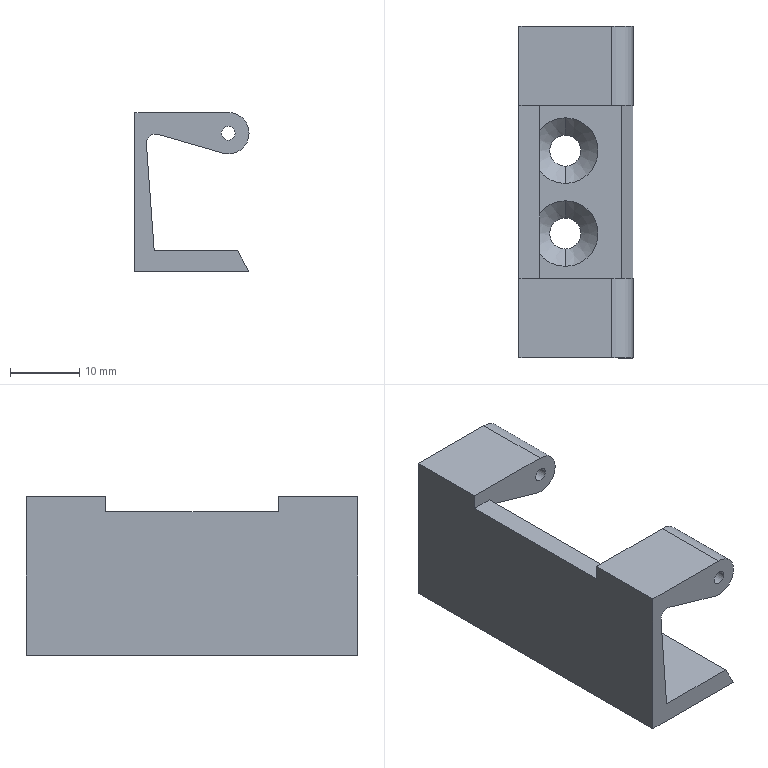Component | SolidWorks | CL201-M6-1-4 | 1 solid | 32 faces | box 16.5 x 48 x 23 mm | volume 5458 mm3 | plane 15 | cylinder 13 | cone 4 | commonest cylinder face diameters 4.5 x4 2 x4 6 x4 2.707 x1
STEP:
#1=COLOUR_RGB('',0.7922,0.8196,0.9333);
#2=FILL_AREA_STYLE_COLOUR('',#1);
#3=FILL_AREA_STYLE('',(#2));
#4=SURFACE_STYLE_FILL_AREA(#3);
#5=SURFACE_SIDE_STYLE('',(#4));
#6=SURFACE_STYLE_USAGE(.BOTH.,#5);
#7=PRESENTATION_STYLE_ASSIGNMENT((#6));
#8=CARTESIAN_POINT('',(12.006,-1.803,15.275));
#9=VERTEX_POINT('',#8);
#10=CARTESIAN_POINT('',(12.006,-1.626,15.275));
#11=VERTEX_POINT('',#10);
#12=CARTESIAN_POINT('',(12.006,-1.714,15.275));
#13=DIRECTION('',(-0.,-0.,1.));
#14=DIRECTION('',(0.,-1.,0.));
#15=AXIS2_PLACEMENT_3D('',#12,#13,#14);
#16=CIRCLE('',#15,0.08858);
#17=EDGE_CURVE('',#9,#11,#16,.T.);
#18=ORIENTED_EDGE('',*,*,#17,.F.);
#19=CARTESIAN_POINT('',(12.006,-1.901,15.373));
#20=VERTEX_POINT('',#19);
#21=CARTESIAN_POINT('',(12.006,-1.803,15.275));
#22=DIRECTION('',(-0.,-0.7071,0.7071));
#23=VECTOR('',#22,39.37);
#24=LINE('',#21,#23);
#25=EDGE_CURVE('',#9,#20,#24,.T.);
#26=ORIENTED_EDGE('',*,*,#25,.T.);
#27=CARTESIAN_POINT('',(12.006,-1.527,15.373));
#28=VERTEX_POINT('',#27);
#29=CARTESIAN_POINT('',(12.006,-1.714,15.373));
#30=DIRECTION('',(0.,0.,-1.));
#31=DIRECTION('',(0.,-1.,0.));
#32=AXIS2_PLACEMENT_3D('',#29,#30,#31);
#33=CIRCLE('',#32,0.187);
#34=EDGE_CURVE('',#28,#20,#33,.T.);
#35=ORIENTED_EDGE('',*,*,#34,.F.);
#36=CARTESIAN_POINT('',(12.006,-1.626,15.275));
#37=DIRECTION('',(-0.,0.7071,0.7071));
#38=VECTOR('',#37,39.37);
#39=LINE('',#36,#38);
#40=EDGE_CURVE('',#11,#28,#39,.T.);
#41=ORIENTED_EDGE('',*,*,#40,.F.);
#42=EDGE_LOOP('',(#18,#26,#35,#41));
#43=FACE_OUTER_BOUND('',#42,.T.);
#44=CARTESIAN_POINT('',(12.006,-1.714,15.275));
#45=DIRECTION('',(-0.,-0.,1.));
#46=DIRECTION('',(0.,1.,0.));
#47=AXIS2_PLACEMENT_3D('',#44,#45,#46);
#48=CONICAL_SURFACE('',#47,0.08858,0.7854);
#49=ADVANCED_FACE('',(#43),#48,.F.);
#50=CARTESIAN_POINT('',(12.006,-1.33,15.275));
#51=VERTEX_POINT('',#50);
#52=CARTESIAN_POINT('',(12.006,-1.153,15.275));
#53=VERTEX_POINT('',#52);
#54=CARTESIAN_POINT('',(12.006,-1.242,15.275));
#55=DIRECTION('',(-0.,-0.,1.));
#56=DIRECTION('',(0.,-1.,0.));
#57=AXIS2_PLACEMENT_3D('',#54,#55,#56);
#58=CIRCLE('',#57,0.08858);
#59=EDGE_CURVE('',#51,#53,#58,.T.);
#60=ORIENTED_EDGE('',*,*,#59,.F.);
#61=CARTESIAN_POINT('',(12.006,-1.429,15.373));
#62=VERTEX_POINT('',#61);
#63=CARTESIAN_POINT('',(12.006,-1.33,15.275));
#64=DIRECTION('',(-0.,-0.7071,0.7071));
#65=VECTOR('',#64,39.37);
#66=LINE('',#63,#65);
#67=EDGE_CURVE('',#51,#62,#66,.T.);
#68=ORIENTED_EDGE('',*,*,#67,.T.);
#69=CARTESIAN_POINT('',(12.006,-1.055,15.373));
#70=VERTEX_POINT('',#69);
#71=CARTESIAN_POINT('',(12.006,-1.242,15.373));
#72=DIRECTION('',(0.,0.,-1.));
#73=DIRECTION('',(0.,-1.,0.));
#74=AXIS2_PLACEMENT_3D('',#71,#72,#73);
#75=CIRCLE('',#74,0.187);
#76=EDGE_CURVE('',#70,#62,#75,.T.);
#77=ORIENTED_EDGE('',*,*,#76,.F.);
#78=CARTESIAN_POINT('',(12.006,-1.153,15.275));
#79=DIRECTION('',(-0.,0.7071,0.7071));
#80=VECTOR('',#79,39.37);
#81=LINE('',#78,#80);
#82=EDGE_CURVE('',#53,#70,#81,.T.);
#83=ORIENTED_EDGE('',*,*,#82,.F.);
#84=EDGE_LOOP('',(#60,#68,#77,#83));
#85=FACE_OUTER_BOUND('',#84,.T.);
#86=CARTESIAN_POINT('',(12.006,-1.242,15.275));
#87=DIRECTION('',(-0.,-0.,1.));
#88=DIRECTION('',(0.,1.,0.));
#89=AXIS2_PLACEMENT_3D('',#86,#87,#88);
#90=CONICAL_SURFACE('',#89,0.08858,0.7854);
#91=ADVANCED_FACE('',(#85),#90,.F.);
#92=CARTESIAN_POINT('',(12.006,-1.153,15.255));
#93=VERTEX_POINT('',#92);
#94=CARTESIAN_POINT('',(12.006,-1.33,15.255));
#95=VERTEX_POINT('',#94);
#96=CARTESIAN_POINT('',(12.006,-1.242,15.255));
#97=DIRECTION('',(0.,0.,-1.));
#98=DIRECTION('',(0.,1.,0.));
#99=AXIS2_PLACEMENT_3D('',#96,#97,#98);
#100=CIRCLE('',#99,0.08858);
#101=EDGE_CURVE('',#93,#95,#100,.T.);
#102=ORIENTED_EDGE('',*,*,#101,.T.);
#103=CARTESIAN_POINT('',(12.006,-1.33,15.255));
#104=DIRECTION('',(-0.,-0.,1.));
#105=VECTOR('',#104,39.37);
#106=LINE('',#103,#105);
#107=EDGE_CURVE('',#95,#51,#106,.T.);
#108=ORIENTED_EDGE('',*,*,#107,.T.);
#109=ORIENTED_EDGE('',*,*,#59,.T.);
#110=CARTESIAN_POINT('',(12.006,-1.153,15.255));
#111=DIRECTION('',(-0.,-0.,1.));
#112=VECTOR('',#111,39.37);
#113=LINE('',#110,#112);
#114=EDGE_CURVE('',#93,#53,#113,.T.);
#115=ORIENTED_EDGE('',*,*,#114,.F.);
#116=EDGE_LOOP('',(#102,#108,#109,#115));
#117=FACE_OUTER_BOUND('',#116,.T.);
#118=CARTESIAN_POINT('',(12.006,-1.242,15.255));
#119=DIRECTION('',(-0.,-0.,1.));
#120=DIRECTION('',(0.,1.,0.));
#121=AXIS2_PLACEMENT_3D('',#118,#119,#120);
#122=CYLINDRICAL_SURFACE('',#121,0.08858);
#123=ADVANCED_FACE('',(#117),#122,.F.);
#124=CARTESIAN_POINT('',(12.006,-1.626,15.255));
#125=VERTEX_POINT('',#124);
#126=CARTESIAN_POINT('',(12.006,-1.803,15.255));
#127=VERTEX_POINT('',#126);
#128=CARTESIAN_POINT('',(12.006,-1.714,15.255));
#129=DIRECTION('',(0.,0.,-1.));
#130=DIRECTION('',(0.,1.,0.));
#131=AXIS2_PLACEMENT_3D('',#128,#129,#130);
#132=CIRCLE('',#131,0.08858);
#133=EDGE_CURVE('',#125,#127,#132,.T.);
#134=ORIENTED_EDGE('',*,*,#133,.T.);
#135=CARTESIAN_POINT('',(12.006,-1.803,15.255));
#136=DIRECTION('',(-0.,-0.,1.));
#137=VECTOR('',#136,39.37);
#138=LINE('',#135,#137);
#139=EDGE_CURVE('',#127,#9,#138,.T.);
#140=ORIENTED_EDGE('',*,*,#139,.T.);
#141=ORIENTED_EDGE('',*,*,#17,.T.);
#142=CARTESIAN_POINT('',(12.006,-1.626,15.255));
#143=DIRECTION('',(-0.,-0.,1.));
#144=VECTOR('',#143,39.37);
#145=LINE('',#142,#144);
#146=EDGE_CURVE('',#125,#11,#145,.T.);
#147=ORIENTED_EDGE('',*,*,#146,.F.);
#148=EDGE_LOOP('',(#134,#140,#141,#147));
#149=FACE_OUTER_BOUND('',#148,.T.);
#150=CARTESIAN_POINT('',(12.006,-1.714,15.255));
#151=DIRECTION('',(-0.,-0.,1.));
#152=DIRECTION('',(0.,1.,0.));
#153=AXIS2_PLACEMENT_3D('',#150,#151,#152);
#154=CYLINDRICAL_SURFACE('',#153,0.08858);
#155=ADVANCED_FACE('',(#149),#154,.F.);
#156=CARTESIAN_POINT('',(12.234,-1.97,16.042));
#157=VERTEX_POINT('',#156);
#158=CARTESIAN_POINT('',(12.313,-1.97,16.042));
#159=VERTEX_POINT('',#158);
#160=CARTESIAN_POINT('',(12.273,-1.97,16.042));
#161=DIRECTION('',(-0.,-1.,-0.));
#162=DIRECTION('',(1.,0.,0.));
#163=AXIS2_PLACEMENT_3D('',#160,#161,#162);
#164=CIRCLE('',#163,0.03937);
#165=EDGE_CURVE('',#157,#159,#164,.T.);
#166=ORIENTED_EDGE('',*,*,#165,.F.);
#167=CARTESIAN_POINT('',(12.234,-2.423,16.042));
#168=VERTEX_POINT('',#167);
#169=CARTESIAN_POINT('',(12.234,-0.5331,16.042));
#170=DIRECTION('',(-0.,-1.,-0.));
#171=VECTOR('',#170,39.37);
#172=LINE('',#169,#171);
#173=EDGE_CURVE('',#157,#168,#172,.T.);
#174=ORIENTED_EDGE('',*,*,#173,.T.);
#175=CARTESIAN_POINT('',(12.313,-2.423,16.042));
#176=VERTEX_POINT('',#175);
#177=CARTESIAN_POINT('',(12.273,-2.423,16.042));
#178=DIRECTION('',(0.,1.,0.));
#179=DIRECTION('',(-1.,0.,0.));
#180=AXIS2_PLACEMENT_3D('',#177,#178,#179);
#181=CIRCLE('',#180,0.03937);
#182=EDGE_CURVE('',#176,#168,#181,.T.);
#183=ORIENTED_EDGE('',*,*,#182,.F.);
#184=CARTESIAN_POINT('',(12.313,-0.5331,16.042));
#185=DIRECTION('',(-0.,-1.,-0.));
#186=VECTOR('',#185,39.37);
#187=LINE('',#184,#186);
#188=EDGE_CURVE('',#159,#176,#187,.T.);
#189=ORIENTED_EDGE('',*,*,#188,.F.);
#190=EDGE_LOOP('',(#166,#174,#183,#189));
#191=FACE_OUTER_BOUND('',#190,.T.);
#192=CARTESIAN_POINT('',(12.273,-0.5331,16.042));
#193=DIRECTION('',(-0.,-1.,-0.));
#194=DIRECTION('',(1.,-0.,0.));
#195=AXIS2_PLACEMENT_3D('',#192,#193,#194);
#196=CYLINDRICAL_SURFACE('',#195,0.03937);
#197=ADVANCED_FACE('',(#191),#196,.F.);
#198=CARTESIAN_POINT('',(12.313,-0.5331,16.042));
#199=VERTEX_POINT('',#198);
#200=CARTESIAN_POINT('',(12.234,-0.5331,16.042));
#201=VERTEX_POINT('',#200);
#202=CARTESIAN_POINT('',(12.273,-0.5331,16.042));
#203=DIRECTION('',(0.,1.,0.));
#204=DIRECTION('',(-1.,0.,0.));
#205=AXIS2_PLACEMENT_3D('',#202,#203,#204);
#206=CIRCLE('',#205,0.03937);
#207=EDGE_CURVE('',#199,#201,#206,.T.);
#208=ORIENTED_EDGE('',*,*,#207,.T.);
#209=CARTESIAN_POINT('',(12.234,-0.9858,16.042));
#210=VERTEX_POINT('',#209);
#211=CARTESIAN_POINT('',(12.234,-0.5331,16.042));
#212=DIRECTION('',(-0.,-1.,-0.));
#213=VECTOR('',#212,39.37);
#214=LINE('',#211,#213);
#215=EDGE_CURVE('',#201,#210,#214,.T.);
#216=ORIENTED_EDGE('',*,*,#215,.T.);
#217=CARTESIAN_POINT('',(12.313,-0.9858,16.042));
#218=VERTEX_POINT('',#217);
#219=CARTESIAN_POINT('',(12.273,-0.9858,16.042));
#220=DIRECTION('',(0.,1.,0.));
#221=DIRECTION('',(-1.,0.,0.));
#222=AXIS2_PLACEMENT_3D('',#219,#220,#221);
#223=CIRCLE('',#222,0.03937);
#224=EDGE_CURVE('',#218,#210,#223,.T.);
#225=ORIENTED_EDGE('',*,*,#224,.F.);
#226=CARTESIAN_POINT('',(12.313,-0.5331,16.042));
#227=DIRECTION('',(-0.,-1.,-0.));
#228=VECTOR('',#227,39.37);
#229=LINE('',#226,#228);
#230=EDGE_CURVE('',#199,#218,#229,.T.);
#231=ORIENTED_EDGE('',*,*,#230,.F.);
#232=EDGE_LOOP('',(#208,#216,#225,#231));
#233=FACE_OUTER_BOUND('',#232,.T.);
#234=CARTESIAN_POINT('',(12.273,-0.5331,16.042));
#235=DIRECTION('',(-0.,-1.,-0.));
#236=DIRECTION('',(1.,-0.,0.));
#237=AXIS2_PLACEMENT_3D('',#234,#235,#236);
#238=CYLINDRICAL_SURFACE('',#237,0.03937);
#239=ADVANCED_FACE('',(#233),#238,.F.);
#240=CARTESIAN_POINT('',(12.251,-1.97,15.926));
#241=VERTEX_POINT('',#240);
#242=CARTESIAN_POINT('',(12.391,-1.97,16.042));
#243=VERTEX_POINT('',#242);
#244=CARTESIAN_POINT('',(12.273,-1.97,16.042));
#245=DIRECTION('',(-0.,-1.,-0.));
#246=DIRECTION('',(1.,-0.,0.));
#247=AXIS2_PLACEMENT_3D('',#244,#245,#246);
#248=CIRCLE('',#247,0.1181);
#249=EDGE_CURVE('',#241,#243,#248,.T.);
#250=ORIENTED_EDGE('',*,*,#249,.T.);
#251=CARTESIAN_POINT('',(12.391,-2.423,16.042));
#252=VERTEX_POINT('',#251);
#253=CARTESIAN_POINT('',(12.391,-0.5331,16.042));
#254=DIRECTION('',(-0.,-1.,-0.));
#255=VECTOR('',#254,39.37);
#256=LINE('',#253,#255);
#257=EDGE_CURVE('',#243,#252,#256,.T.);
#258=ORIENTED_EDGE('',*,*,#257,.T.);
#259=CARTESIAN_POINT('',(12.251,-2.423,15.926));
#260=VERTEX_POINT('',#259);
#261=CARTESIAN_POINT('',(12.273,-2.423,16.042));
#262=DIRECTION('',(0.,1.,0.));
#263=DIRECTION('',(-1.,0.,-0.));
#264=AXIS2_PLACEMENT_3D('',#261,#262,#263);
#265=CIRCLE('',#264,0.1181);
#266=EDGE_CURVE('',#252,#260,#265,.T.);
#267=ORIENTED_EDGE('',*,*,#266,.T.);
#268=CARTESIAN_POINT('',(12.251,-0.5331,15.926));
#269=DIRECTION('',(-0.,-1.,-0.));
#270=VECTOR('',#269,39.37);
#271=LINE('',#268,#270);
#272=EDGE_CURVE('',#241,#260,#271,.T.);
#273=ORIENTED_EDGE('',*,*,#272,.F.);
#274=EDGE_LOOP('',(#250,#258,#267,#273));
#275=FACE_OUTER_BOUND('',#274,.T.);
#276=CARTESIAN_POINT('',(12.273,-0.5331,16.042));
#277=DIRECTION('',(-0.,-1.,-0.));
#278=DIRECTION('',(1.,-0.,0.));
#279=AXIS2_PLACEMENT_3D('',#276,#277,#278);
#280=CYLINDRICAL_SURFACE('',#279,0.1181);
#281=ADVANCED_FACE('',(#275),#280,.T.);
#282=CARTESIAN_POINT('',(12.391,-0.5331,16.042));
#283=VERTEX_POINT('',#282);
#284=CARTESIAN_POINT('',(12.251,-0.5331,15.926));
#285=VERTEX_POINT('',#284);
#286=CARTESIAN_POINT('',(12.273,-0.5331,16.042));
#287=DIRECTION('',(0.,1.,0.));
#288=DIRECTION('',(-1.,0.,-0.));
#289=AXIS2_PLACEMENT_3D('',#286,#287,#288);
#290=CIRCLE('',#289,0.1181);
#291=EDGE_CURVE('',#283,#285,#290,.T.);
#292=ORIENTED_EDGE('',*,*,#291,.F.);
#293=CARTESIAN_POINT('',(12.391,-0.9858,16.042));
#294=VERTEX_POINT('',#293);
#295=CARTESIAN_POINT('',(12.391,-0.5331,16.042));
#296=DIRECTION('',(-0.,-1.,-0.));
#297=VECTOR('',#296,39.37);
#298=LINE('',#295,#297);
#299=EDGE_CURVE('',#283,#294,#298,.T.);
#300=ORIENTED_EDGE('',*,*,#299,.T.);
#301=CARTESIAN_POINT('',(12.251,-0.9858,15.926));
#302=VERTEX_POINT('',#301);
#303=CARTESIAN_POINT('',(12.273,-0.9858,16.042));
#304=DIRECTION('',(0.,1.,0.));
#305=DIRECTION('',(-1.,0.,-0.));
#306=AXIS2_PLACEMENT_3D('',#303,#304,#305);
#307=CIRCLE('',#306,0.1181);
#308=EDGE_CURVE('',#294,#302,#307,.T.);
#309=ORIENTED_EDGE('',*,*,#308,.T.);
#310=CARTESIAN_POINT('',(12.251,-0.5331,15.926));
#311=DIRECTION('',(-0.,-1.,-0.));
#312=VECTOR('',#311,39.37);
#313=LINE('',#310,#312);
#314=EDGE_CURVE('',#285,#302,#313,.T.);
#315=ORIENTED_EDGE('',*,*,#314,.F.);
#316=EDGE_LOOP('',(#292,#300,#309,#315));
#317=FACE_OUTER_BOUND('',#316,.T.);
#318=CARTESIAN_POINT('',(12.273,-0.5331,16.042));
#319=DIRECTION('',(-0.,-1.,-0.));
#320=DIRECTION('',(1.,-0.,0.));
#321=AXIS2_PLACEMENT_3D('',#318,#319,#320);
#322=CYLINDRICAL_SURFACE('',#321,0.1181);
#323=ADVANCED_FACE('',(#317),#322,.T.);
#324=CARTESIAN_POINT('',(11.742,-0.5331,16.16));
#325=VERTEX_POINT('',#324);
#326=CARTESIAN_POINT('',(11.742,-0.9858,16.16));
#327=VERTEX_POINT('',#326);
#328=CARTESIAN_POINT('',(11.742,-0.5331,16.16));
#329=DIRECTION('',(-0.,-1.,-0.));
#330=VECTOR('',#329,39.37);
#331=LINE('',#328,#330);
#332=EDGE_CURVE('',#325,#327,#331,.T.);
#333=ORIENTED_EDGE('',*,*,#332,.T.);
#334=CARTESIAN_POINT('',(12.269,-0.9858,16.16));
#335=VERTEX_POINT('',#334);
#336=CARTESIAN_POINT('',(11.86,-0.9858,16.16));
#337=DIRECTION('',(-1.,0.,-0.));
#338=VECTOR('',#337,39.37);
#339=LINE('',#336,#338);
#340=EDGE_CURVE('',#335,#327,#339,.T.);
#341=ORIENTED_EDGE('',*,*,#340,.F.);
#342=CARTESIAN_POINT('',(12.269,-0.5331,16.16));
#343=VERTEX_POINT('',#342);
#344=CARTESIAN_POINT('',(12.269,-0.5331,16.16));
#345=DIRECTION('',(-0.,-1.,-0.));
#346=VECTOR('',#345,39.37);
#347=LINE('',#344,#346);
#348=EDGE_CURVE('',#343,#335,#347,.T.);
#349=ORIENTED_EDGE('',*,*,#348,.F.);
#350=CARTESIAN_POINT('',(12.269,-0.5331,16.16));
#351=DIRECTION('',(1.,-0.,0.));
#352=VECTOR('',#351,39.37);
#353=LINE('',#350,#352);
#354=EDGE_CURVE('',#325,#343,#353,.T.);
#355=ORIENTED_EDGE('',*,*,#354,.F.);
#356=EDGE_LOOP('',(#333,#341,#349,#355));
#357=FACE_OUTER_BOUND('',#356,.T.);
#358=CARTESIAN_POINT('',(12.269,-0.5331,16.16));
#359=DIRECTION('',(0.,0.,-1.));
#360=DIRECTION('',(-0.,-1.,-0.));
#361=AXIS2_PLACEMENT_3D('',#358,#359,#360);
#362=PLANE('',#361);
#363=ADVANCED_FACE('',(#357),#362,.F.);
#364=CARTESIAN_POINT('',(11.742,-1.97,16.16));
#365=VERTEX_POINT('',#364);
#366=CARTESIAN_POINT('',(12.269,-1.97,16.16));
#367=VERTEX_POINT('',#366);
#368=CARTESIAN_POINT('',(11.86,-1.97,16.16));
#369=DIRECTION('',(1.,-0.,0.));
#370=VECTOR('',#369,39.37);
#371=LINE('',#368,#370);
#372=EDGE_CURVE('',#365,#367,#371,.T.);
#373=ORIENTED_EDGE('',*,*,#372,.F.);
#374=CARTESIAN_POINT('',(11.742,-2.423,16.16));
#375=VERTEX_POINT('',#374);
#376=CARTESIAN_POINT('',(11.742,-0.5331,16.16));
#377=DIRECTION('',(-0.,-1.,-0.));
#378=VECTOR('',#377,39.37);
#379=LINE('',#376,#378);
#380=EDGE_CURVE('',#365,#375,#379,.T.);
#381=ORIENTED_EDGE('',*,*,#380,.T.);
#382=CARTESIAN_POINT('',(12.269,-2.423,16.16));
#383=VERTEX_POINT('',#382);
#384=CARTESIAN_POINT('',(12.269,-2.423,16.16));
#385=DIRECTION('',(1.,-0.,0.));
#386=VECTOR('',#385,39.37);
#387=LINE('',#384,#386);
#388=EDGE_CURVE('',#375,#383,#387,.T.);
#389=ORIENTED_EDGE('',*,*,#388,.T.);
#390=CARTESIAN_POINT('',(12.269,-0.5331,16.16));
#391=DIRECTION('',(-0.,-1.,-0.));
#392=VECTOR('',#391,39.37);
#393=LINE('',#390,#392);
#394=EDGE_CURVE('',#367,#383,#393,.T.);
#395=ORIENTED_EDGE('',*,*,#394,.F.);
#396=EDGE_LOOP('',(#373,#381,#389,#395));
#397=FACE_OUTER_BOUND('',#396,.T.);
#398=CARTESIAN_POINT('',(12.269,-0.5331,16.16));
#399=DIRECTION('',(0.,0.,-1.));
#400=DIRECTION('',(-0.,-1.,-0.));
#401=AXIS2_PLACEMENT_3D('',#398,#399,#400);
#402=PLANE('',#401);
#403=ADVANCED_FACE('',(#397),#402,.F.);
#404=CARTESIAN_POINT('',(11.86,-1.97,16.074));
#405=VERTEX_POINT('',#404);
#406=CARTESIAN_POINT('',(11.86,-0.9858,16.074));
#407=VERTEX_POINT('',#406);
#408=CARTESIAN_POINT('',(11.86,-1.97,16.074));
#409=DIRECTION('',(0.,1.,0.));
#410=VECTOR('',#409,39.37);
#411=LINE('',#408,#410);
#412=EDGE_CURVE('',#405,#407,#411,.T.);
#413=ORIENTED_EDGE('',*,*,#412,.F.);
#414=CARTESIAN_POINT('',(11.86,-1.97,16.038));
#415=VERTEX_POINT('',#414);
#416=CARTESIAN_POINT('',(11.86,-1.97,14.246));
#417=DIRECTION('',(-0.,-0.,1.));
#418=VECTOR('',#417,39.37);
#419=LINE('',#416,#418);
#420=EDGE_CURVE('',#415,#405,#419,.T.);
#421=ORIENTED_EDGE('',*,*,#420,.F.);
#422=CARTESIAN_POINT('',(11.86,-0.9858,16.038));
#423=VERTEX_POINT('',#422);
#424=CARTESIAN_POINT('',(11.86,-0.5331,16.038));
#425=DIRECTION('',(-0.,-1.,-0.));
#426=VECTOR('',#425,39.37);
#427=LINE('',#424,#426);
#428=EDGE_CURVE('',#423,#415,#427,.T.);
#429=ORIENTED_EDGE('',*,*,#428,.F.);
#430=CARTESIAN_POINT('',(11.86,-0.9858,14.246));
#431=DIRECTION('',(-0.,-0.,1.));
#432=VECTOR('',#431,39.37);
#433=LINE('',#430,#432);
#434=EDGE_CURVE('',#423,#407,#433,.T.);
#435=ORIENTED_EDGE('',*,*,#434,.T.);
#436=EDGE_LOOP('',(#413,#421,#429,#435));
#437=FACE_OUTER_BOUND('',#436,.T.);
#438=CARTESIAN_POINT('',(11.86,-1.97,14.246));
#439=DIRECTION('',(-1.,0.,-0.));
#440=DIRECTION('',(-0.,-1.,-0.));
#441=AXIS2_PLACEMENT_3D('',#438,#439,#440);
#442=PLANE('',#441);
#443=ADVANCED_FACE('',(#437),#442,.F.);
#444=ORIENTED_EDGE('',*,*,#299,.F.);
#445=CARTESIAN_POINT('',(12.273,-0.5331,16.042));
#446=DIRECTION('',(0.,1.,0.));
#447=DIRECTION('',(-1.,0.,-0.));
#448=AXIS2_PLACEMENT_3D('',#445,#446,#447);
#449=CIRCLE('',#448,0.1181);
#450=EDGE_CURVE('',#343,#283,#449,.T.);
#451=ORIENTED_EDGE('',*,*,#450,.F.);
#452=ORIENTED_EDGE('',*,*,#348,.T.);
#453=CARTESIAN_POINT('',(12.273,-0.9858,16.042));
#454=DIRECTION('',(0.,1.,0.));
#455=DIRECTION('',(-1.,0.,-0.));
#456=AXIS2_PLACEMENT_3D('',#453,#454,#455);
#457=CIRCLE('',#456,0.1181);
#458=EDGE_CURVE('',#335,#294,#457,.T.);
#459=ORIENTED_EDGE('',*,*,#458,.T.);
#460=EDGE_LOOP('',(#444,#451,#452,#459));
#461=FACE_OUTER_BOUND('',#460,.T.);
#462=CARTESIAN_POINT('',(12.273,-0.5331,16.042));
#463=DIRECTION('',(-0.,-1.,-0.));
#464=DIRECTION('',(1.,-0.,0.));
#465=AXIS2_PLACEMENT_3D('',#462,#463,#464);
#466=CYLINDRICAL_SURFACE('',#465,0.1181);
#467=ADVANCED_FACE('',(#461),#466,.T.);
#468=ORIENTED_EDGE('',*,*,#257,.F.);
#469=CARTESIAN_POINT('',(12.273,-1.97,16.042));
#470=DIRECTION('',(-0.,-1.,-0.));
#471=DIRECTION('',(1.,-0.,0.));
#472=AXIS2_PLACEMENT_3D('',#469,#470,#471);
#473=CIRCLE('',#472,0.1181);
#474=EDGE_CURVE('',#243,#367,#473,.T.);
#475=ORIENTED_EDGE('',*,*,#474,.T.);
#476=ORIENTED_EDGE('',*,*,#394,.T.);
#477=CARTESIAN_POINT('',(12.273,-2.423,16.042));
#478=DIRECTION('',(0.,1.,0.));
#479=DIRECTION('',(-1.,0.,-0.));
#480=AXIS2_PLACEMENT_3D('',#477,#478,#479);
#481=CIRCLE('',#480,0.1181);
#482=EDGE_CURVE('',#383,#252,#481,.T.);
#483=ORIENTED_EDGE('',*,*,#482,.T.);
#484=EDGE_LOOP('',(#468,#475,#476,#483));
#485=FACE_OUTER_BOUND('',#484,.T.);
#486=CARTESIAN_POINT('',(12.273,-0.5331,16.042));
#487=DIRECTION('',(-0.,-1.,-0.));
#488=DIRECTION('',(1.,-0.,0.));
#489=AXIS2_PLACEMENT_3D('',#486,#487,#488);
#490=CYLINDRICAL_SURFACE('',#489,0.1181);
#491=ADVANCED_FACE('',(#485),#490,.T.);
#492=ORIENTED_EDGE('',*,*,#314,.T.);
#493=CARTESIAN_POINT('',(11.875,-0.9858,16.035));
#494=VERTEX_POINT('',#493);
#495=CARTESIAN_POINT('',(12.251,-0.9858,15.926));
#496=DIRECTION('',(-0.9604,0.,0.2785));
#497=VECTOR('',#496,39.37);
#498=LINE('',#495,#497);
#499=EDGE_CURVE('',#302,#494,#498,.T.);
#500=ORIENTED_EDGE('',*,*,#499,.T.);
#501=CARTESIAN_POINT('',(11.875,-0.5331,16.035));
#502=VERTEX_POINT('',#501);
#503=CARTESIAN_POINT('',(11.875,-0.5331,16.035));
#504=DIRECTION('',(-0.,-1.,-0.));
#505=VECTOR('',#504,39.37);
#506=LINE('',#503,#505);
#507=EDGE_CURVE('',#502,#494,#506,.T.);
#508=ORIENTED_EDGE('',*,*,#507,.F.);
#509=CARTESIAN_POINT('',(12.251,-0.5331,15.926));
#510=DIRECTION('',(-0.9604,0.,0.2785));
#511=VECTOR('',#510,39.37);
#512=LINE('',#509,#511);
#513=EDGE_CURVE('',#285,#502,#512,.T.);
#514=ORIENTED_EDGE('',*,*,#513,.F.);
#515=EDGE_LOOP('',(#492,#500,#508,#514));
#516=FACE_OUTER_BOUND('',#515,.T.);
#517=CARTESIAN_POINT('',(12.251,-0.5331,15.926));
#518=DIRECTION('',(0.2785,-0.,0.9604));
#519=DIRECTION('',(0.9604,-0.,-0.2785));
#520=AXIS2_PLACEMENT_3D('',#517,#518,#519);
#521=PLANE('',#520);
#522=ADVANCED_FACE('',(#516),#521,.F.);
#523=ORIENTED_EDGE('',*,*,#215,.F.);
#524=CARTESIAN_POINT('',(12.273,-0.5331,16.042));
#525=DIRECTION('',(0.,1.,0.));
#526=DIRECTION('',(-1.,0.,0.));
#527=AXIS2_PLACEMENT_3D('',#524,#525,#526);
#528=CIRCLE('',#527,0.03937);
#529=EDGE_CURVE('',#201,#199,#528,.T.);
#530=ORIENTED_EDGE('',*,*,#529,.T.);
#531=ORIENTED_EDGE('',*,*,#230,.T.);
#532=CARTESIAN_POINT('',(12.273,-0.9858,16.042));
#533=DIRECTION('',(0.,1.,0.));
#534=DIRECTION('',(-1.,0.,0.));
#535=AXIS2_PLACEMENT_3D('',#532,#533,#534);
#536=CIRCLE('',#535,0.03937);
#537=EDGE_CURVE('',#210,#218,#536,.T.);
#538=ORIENTED_EDGE('',*,*,#537,.F.);
#539=EDGE_LOOP('',(#523,#530,#531,#538));
#540=FACE_OUTER_BOUND('',#539,.T.);
#541=CARTESIAN_POINT('',(12.273,-0.5331,16.042));
#542=DIRECTION('',(-0.,-1.,-0.));
#543=DIRECTION('',(1.,-0.,0.));
#544=AXIS2_PLACEMENT_3D('',#541,#542,#543);
#545=CYLINDRICAL_SURFACE('',#544,0.03937);
#546=ADVANCED_FACE('',(#540),#545,.F.);
#547=CARTESIAN_POINT('',(11.742,-0.5331,15.255));
#548=VERTEX_POINT('',#547);
#549=CARTESIAN_POINT('',(11.742,-0.5331,16.16));
#550=DIRECTION('',(-0.,-0.,1.));
#551=VECTOR('',#550,39.37);
#552=LINE('',#549,#551);
#553=EDGE_CURVE('',#548,#325,#552,.T.);
#554=ORIENTED_EDGE('',*,*,#553,.T.);
#555=ORIENTED_EDGE('',*,*,#354,.T.);
#556=ORIENTED_EDGE('',*,*,#450,.T.);
#557=ORIENTED_EDGE('',*,*,#291,.T.);
#558=ORIENTED_EDGE('',*,*,#513,.T.);
#559=CARTESIAN_POINT('',(11.807,-0.5331,15.984));
#560=VERTEX_POINT('',#559);
#561=CARTESIAN_POINT('',(11.86,-0.5331,15.984));
#562=DIRECTION('',(-0.,-1.,-0.));
#563=DIRECTION('',(-1.,0.,0.));
#564=AXIS2_PLACEMENT_3D('',#561,#562,#563);
#565=CIRCLE('',#564,0.05329);
#566=EDGE_CURVE('',#502,#560,#565,.T.);
#567=ORIENTED_EDGE('',*,*,#566,.T.);
#568=CARTESIAN_POINT('',(11.851,-0.5331,15.373));
#569=VERTEX_POINT('',#568);
#570=CARTESIAN_POINT('',(11.807,-0.5331,15.984));
#571=DIRECTION('',(0.07258,-0.,-0.9974));
#572=VECTOR('',#571,39.37);
#573=LINE('',#570,#572);
#574=EDGE_CURVE('',#560,#569,#573,.T.);
#575=ORIENTED_EDGE('',*,*,#574,.T.);
#576=CARTESIAN_POINT('',(12.326,-0.5331,15.373));
#577=VERTEX_POINT('',#576);
#578=CARTESIAN_POINT('',(12.326,-0.5331,15.373));
#579=DIRECTION('',(1.,-0.,0.));
#580=VECTOR('',#579,39.37);
#581=LINE('',#578,#580);
#582=EDGE_CURVE('',#569,#577,#581,.T.);
#583=ORIENTED_EDGE('',*,*,#582,.T.);
#584=CARTESIAN_POINT('',(12.391,-0.5331,15.255));
#585=VERTEX_POINT('',#584);
#586=CARTESIAN_POINT('',(12.391,-0.5331,15.255));
#587=DIRECTION('',(0.4829,-0.,-0.8757));
#588=VECTOR('',#587,39.37);
#589=LINE('',#586,#588);
#590=EDGE_CURVE('',#577,#585,#589,.T.);
#591=ORIENTED_EDGE('',*,*,#590,.T.);
#592=CARTESIAN_POINT('',(12.391,-0.5331,15.255));
#593=DIRECTION('',(-1.,0.,-0.));
#594=VECTOR('',#593,39.37);
#595=LINE('',#592,#594);
#596=EDGE_CURVE('',#585,#548,#595,.T.);
#597=ORIENTED_EDGE('',*,*,#596,.T.);
#598=EDGE_LOOP('',(#554,#555,#556,#557,#558,#567,#575,#583,#591,#597));
#599=FACE_OUTER_BOUND('',#598,.T.);
#600=ORIENTED_EDGE('',*,*,#207,.F.);
#601=ORIENTED_EDGE('',*,*,#529,.F.);
#602=EDGE_LOOP('',(#600,#601));
#603=FACE_BOUND('',#602,.T.);
#604=CARTESIAN_POINT('',(11.86,-0.5331,15.984));
#605=DIRECTION('',(0.,1.,0.));
#606=DIRECTION('',(-1.,0.,-0.));
#607=AXIS2_PLACEMENT_3D('',#604,#605,#606);
#608=PLANE('',#607);
#609=ADVANCED_FACE('',(#599,#603),#608,.T.);
#610=CARTESIAN_POINT('',(11.742,-2.423,15.255));
#611=VERTEX_POINT('',#610);
#612=CARTESIAN_POINT('',(11.742,-2.423,16.16));
#613=DIRECTION('',(-0.,-0.,1.));
#614=VECTOR('',#613,39.37);
#615=LINE('',#612,#614);
#616=EDGE_CURVE('',#611,#375,#615,.T.);
#617=ORIENTED_EDGE('',*,*,#616,.F.);
#618=CARTESIAN_POINT('',(12.391,-2.423,15.255));
#619=VERTEX_POINT('',#618);
#620=CARTESIAN_POINT('',(12.391,-2.423,15.255));
#621=DIRECTION('',(-1.,0.,-0.));
#622=VECTOR('',#621,39.37);
#623=LINE('',#620,#622);
#624=EDGE_CURVE('',#619,#611,#623,.T.);
#625=ORIENTED_EDGE('',*,*,#624,.F.);
#626=CARTESIAN_POINT('',(12.326,-2.423,15.373));
#627=VERTEX_POINT('',#626);
#628=CARTESIAN_POINT('',(12.391,-2.423,15.255));
#629=DIRECTION('',(0.4829,-0.,-0.8757));
#630=VECTOR('',#629,39.37);
#631=LINE('',#628,#630);
#632=EDGE_CURVE('',#627,#619,#631,.T.);
#633=ORIENTED_EDGE('',*,*,#632,.F.);
#634=CARTESIAN_POINT('',(11.851,-2.423,15.373));
#635=VERTEX_POINT('',#634);
#636=CARTESIAN_POINT('',(12.326,-2.423,15.373));
#637=DIRECTION('',(1.,-0.,0.));
#638=VECTOR('',#637,39.37);
#639=LINE('',#636,#638);
#640=EDGE_CURVE('',#635,#627,#639,.T.);
#641=ORIENTED_EDGE('',*,*,#640,.F.);
#642=CARTESIAN_POINT('',(11.807,-2.423,15.984));
#643=VERTEX_POINT('',#642);
#644=CARTESIAN_POINT('',(11.807,-2.423,15.984));
#645=DIRECTION('',(0.07258,-0.,-0.9974));
#646=VECTOR('',#645,39.37);
#647=LINE('',#644,#646);
#648=EDGE_CURVE('',#643,#635,#647,.T.);
#649=ORIENTED_EDGE('',*,*,#648,.F.);
#650=CARTESIAN_POINT('',(11.875,-2.423,16.035));
#651=VERTEX_POINT('',#650);
#652=CARTESIAN_POINT('',(11.86,-2.423,15.984));
#653=DIRECTION('',(-0.,-1.,-0.));
#654=DIRECTION('',(-1.,0.,0.));
#655=AXIS2_PLACEMENT_3D('',#652,#653,#654);
#656=CIRCLE('',#655,0.05329);
#657=EDGE_CURVE('',#651,#643,#656,.T.);
#658=ORIENTED_EDGE('',*,*,#657,.F.);
#659=CARTESIAN_POINT('',(12.251,-2.423,15.926));
#660=DIRECTION('',(-0.9604,0.,0.2785));
#661=VECTOR('',#660,39.37);
#662=LINE('',#659,#661);
#663=EDGE_CURVE('',#260,#651,#662,.T.);
#664=ORIENTED_EDGE('',*,*,#663,.F.);
#665=ORIENTED_EDGE('',*,*,#266,.F.);
#666=ORIENTED_EDGE('',*,*,#482,.F.);
#667=ORIENTED_EDGE('',*,*,#388,.F.);
#668=EDGE_LOOP('',(#617,#625,#633,#641,#649,#658,#664,#665,#666,#667));
#669=FACE_OUTER_BOUND('',#668,.T.);
#670=ORIENTED_EDGE('',*,*,#182,.T.);
#671=CARTESIAN_POINT('',(12.273,-2.423,16.042));
#672=DIRECTION('',(0.,1.,0.));
#673=DIRECTION('',(-1.,0.,0.));
#674=AXIS2_PLACEMENT_3D('',#671,#672,#673);
#675=CIRCLE('',#674,0.03937);
#676=EDGE_CURVE('',#168,#176,#675,.T.);
#677=ORIENTED_EDGE('',*,*,#676,.T.);
#678=EDGE_LOOP('',(#670,#677));
#679=FACE_BOUND('',#678,.T.);
#680=CARTESIAN_POINT('',(11.86,-2.423,15.984));
#681=DIRECTION('',(0.,1.,0.));
#682=DIRECTION('',(-1.,0.,-0.));
#683=AXIS2_PLACEMENT_3D('',#680,#681,#682);
#684=PLANE('',#683);
#685=ADVANCED_FACE('',(#669,#679),#684,.F.);
#686=ORIENTED_EDGE('',*,*,#380,.F.);
#687=CARTESIAN_POINT('',(11.742,-1.97,16.074));
#688=VERTEX_POINT('',#687);
#689=CARTESIAN_POINT('',(11.742,-1.97,16.16));
#690=DIRECTION('',(0.,-0.,-1.));
#691=VECTOR('',#690,39.37);
#692=LINE('',#689,#691);
#693=EDGE_CURVE('',#365,#688,#692,.T.);
#694=ORIENTED_EDGE('',*,*,#693,.T.);
#695=CARTESIAN_POINT('',(11.742,-0.9858,16.074));
#696=VERTEX_POINT('',#695);
#697=CARTESIAN_POINT('',(11.742,-0.5331,16.074));
#698=DIRECTION('',(-0.,-1.,-0.));
#699=VECTOR('',#698,39.37);
#700=LINE('',#697,#699);
#701=EDGE_CURVE('',#696,#688,#700,.T.);
#702=ORIENTED_EDGE('',*,*,#701,.F.);
#703=CARTESIAN_POINT('',(11.742,-0.9858,16.16));
#704=DIRECTION('',(-0.,0.,1.));
#705=VECTOR('',#704,39.37);
#706=LINE('',#703,#705);
#707=EDGE_CURVE('',#696,#327,#706,.T.);
#708=ORIENTED_EDGE('',*,*,#707,.T.);
#709=ORIENTED_EDGE('',*,*,#332,.F.);
#710=ORIENTED_EDGE('',*,*,#553,.F.);
#711=CARTESIAN_POINT('',(11.742,-0.5331,15.255));
#712=DIRECTION('',(-0.,-1.,-0.));
#713=VECTOR('',#712,39.37);
#714=LINE('',#711,#713);
#715=EDGE_CURVE('',#548,#611,#714,.T.);
#716=ORIENTED_EDGE('',*,*,#715,.T.);
#717=ORIENTED_EDGE('',*,*,#616,.T.);
#718=EDGE_LOOP('',(#686,#694,#702,#708,#709,#710,#716,#717));
#719=FACE_OUTER_BOUND('',#718,.T.);
#720=CARTESIAN_POINT('',(11.742,-0.5331,16.16));
#721=DIRECTION('',(1.,-0.,0.));
#722=DIRECTION('',(0.,0.,-1.));
#723=AXIS2_PLACEMENT_3D('',#720,#721,#722);
#724=PLANE('',#723);
#725=ADVANCED_FACE('',(#719),#724,.F.);
#726=CARTESIAN_POINT('',(11.875,-1.97,16.035));
#727=VERTEX_POINT('',#726);
#728=CARTESIAN_POINT('',(11.875,-0.5331,16.035));
#729=DIRECTION('',(-0.,-1.,-0.));
#730=VECTOR('',#729,39.37);
#731=LINE('',#728,#730);
#732=EDGE_CURVE('',#727,#651,#731,.T.);
#733=ORIENTED_EDGE('',*,*,#732,.F.);
#734=CARTESIAN_POINT('',(12.251,-1.97,15.926));
#735=DIRECTION('',(0.9604,-0.,-0.2785));
#736=VECTOR('',#735,39.37);
#737=LINE('',#734,#736);
#738=EDGE_CURVE('',#727,#241,#737,.T.);
#739=ORIENTED_EDGE('',*,*,#738,.T.);
#740=ORIENTED_EDGE('',*,*,#272,.T.);
#741=ORIENTED_EDGE('',*,*,#663,.T.);
#742=EDGE_LOOP('',(#733,#739,#740,#741));
#743=FACE_OUTER_BOUND('',#742,.T.);
#744=CARTESIAN_POINT('',(12.251,-0.5331,15.926));
#745=DIRECTION('',(0.2785,-0.,0.9604));
#746=DIRECTION('',(0.9604,-0.,-0.2785));
#747=AXIS2_PLACEMENT_3D('',#744,#745,#746);
#748=PLANE('',#747);
#749=ADVANCED_FACE('',(#743),#748,.F.);
#750=ORIENTED_EDGE('',*,*,#507,.T.);
#751=CARTESIAN_POINT('',(11.86,-0.9858,15.984));
#752=DIRECTION('',(-0.,-1.,-0.));
#753=DIRECTION('',(-1.,0.,-0.));
#754=AXIS2_PLACEMENT_3D('',#751,#752,#753);
#755=CIRCLE('',#754,0.05329);
#756=EDGE_CURVE('',#494,#423,#755,.T.);
#757=ORIENTED_EDGE('',*,*,#756,.T.);
#758=ORIENTED_EDGE('',*,*,#428,.T.);
#759=CARTESIAN_POINT('',(11.86,-1.97,15.984));
#760=DIRECTION('',(0.,1.,0.));
#761=DIRECTION('',(1.,0.,-0.));
#762=AXIS2_PLACEMENT_3D('',#759,#760,#761);
#763=CIRCLE('',#762,0.05329);
#764=EDGE_CURVE('',#415,#727,#763,.T.);
#765=ORIENTED_EDGE('',*,*,#764,.T.);
#766=ORIENTED_EDGE('',*,*,#732,.T.);
#767=ORIENTED_EDGE('',*,*,#657,.T.);
#768=CARTESIAN_POINT('',(11.807,-0.5331,15.984));
#769=DIRECTION('',(-0.,-1.,-0.));
#770=VECTOR('',#769,39.37);
#771=LINE('',#768,#770);
#772=EDGE_CURVE('',#560,#643,#771,.T.);
#773=ORIENTED_EDGE('',*,*,#772,.F.);
#774=ORIENTED_EDGE('',*,*,#566,.F.);
#775=EDGE_LOOP('',(#750,#757,#758,#765,#766,#767,#773,#774));
#776=FACE_OUTER_BOUND('',#775,.T.);
#777=CARTESIAN_POINT('',(11.86,-0.5331,15.984));
#778=DIRECTION('',(-0.,-1.,-0.));
#779=DIRECTION('',(1.,-0.,0.));
#780=AXIS2_PLACEMENT_3D('',#777,#778,#779);
#781=CYLINDRICAL_SURFACE('',#780,0.05329);
#782=ADVANCED_FACE('',(#776),#781,.F.);
#783=ORIENTED_EDGE('',*,*,#648,.T.);
#784=CARTESIAN_POINT('',(11.851,-1.82,15.373));
#785=VERTEX_POINT('',#784);
#786=CARTESIAN_POINT('',(11.851,-0.5331,15.373));
#787=DIRECTION('',(-0.,-1.,-0.));
#788=VECTOR('',#787,39.37);
#789=LINE('',#786,#788);
#790=EDGE_CURVE('',#785,#635,#789,.T.);
#791=ORIENTED_EDGE('',*,*,#790,.F.);
#792=CARTESIAN_POINT('',(11.851,-1.609,15.373));
#793=VERTEX_POINT('',#792);
#794=CARTESIAN_POINT('',(11.851,-1.82,15.373));
#795=CARTESIAN_POINT('',(11.852,-1.804,15.363));
#796=CARTESIAN_POINT('',(11.852,-1.787,15.355));
#797=CARTESIAN_POINT('',(11.853,-1.761,15.345));
#798=CARTESIAN_POINT('',(11.853,-1.751,15.342));
#799=CARTESIAN_POINT('',(11.854,-1.733,15.339));
#800=CARTESIAN_POINT('',(11.854,-1.724,15.338));
#801=CARTESIAN_POINT('',(11.854,-1.705,15.338));
#802=CARTESIAN_POINT('',(11.854,-1.696,15.339));
#803=CARTESIAN_POINT('',(11.853,-1.677,15.342));
#804=CARTESIAN_POINT('',(11.853,-1.668,15.345));
#805=CARTESIAN_POINT('',(11.853,-1.65,15.351));
#806=CARTESIAN_POINT('',(11.852,-1.642,15.355));
#807=CARTESIAN_POINT('',(11.852,-1.625,15.364));
#808=CARTESIAN_POINT('',(11.851,-1.617,15.368));
#809=CARTESIAN_POINT('',(11.851,-1.609,15.373));
#810=B_SPLINE_CURVE_WITH_KNOTS('',3,(#794,#795,#796,#797,#798,#799,#800,#801,#802,#803,#804,#805,#806,#807,#808,#809),.UNSPECIFIED.,.F.,.F.,(4,2,2,2,2,2,2,4),(0.,0.001422,0.002132,0.002843,0.003554,0.004265,0.004975,0.005686),.UNSPECIFIED.);
#811=EDGE_CURVE('',#785,#793,#810,.T.);
#812=ORIENTED_EDGE('',*,*,#811,.T.);
#813=CARTESIAN_POINT('',(11.851,-1.347,15.373));
#814=VERTEX_POINT('',#813);
#815=CARTESIAN_POINT('',(11.851,-0.5331,15.373));
#816=DIRECTION('',(-0.,-1.,-0.));
#817=VECTOR('',#816,39.37);
#818=LINE('',#815,#817);
#819=EDGE_CURVE('',#814,#793,#818,.T.);
#820=ORIENTED_EDGE('',*,*,#819,.F.);
#821=CARTESIAN_POINT('',(11.851,-1.136,15.373));
#822=VERTEX_POINT('',#821);
#823=CARTESIAN_POINT('',(11.851,-1.347,15.373));
#824=CARTESIAN_POINT('',(11.852,-1.331,15.363));
#825=CARTESIAN_POINT('',(11.852,-1.314,15.355));
#826=CARTESIAN_POINT('',(11.853,-1.288,15.345));
#827=CARTESIAN_POINT('',(11.853,-1.279,15.342));
#828=CARTESIAN_POINT('',(11.854,-1.261,15.339));
#829=CARTESIAN_POINT('',(11.854,-1.251,15.338));
#830=CARTESIAN_POINT('',(11.854,-1.233,15.338));
#831=CARTESIAN_POINT('',(11.854,-1.223,15.339));
#832=CARTESIAN_POINT('',(11.853,-1.205,15.342));
#833=CARTESIAN_POINT('',(11.853,-1.196,15.345));
#834=CARTESIAN_POINT('',(11.853,-1.178,15.351));
#835=CARTESIAN_POINT('',(11.852,-1.169,15.355));
#836=CARTESIAN_POINT('',(11.852,-1.153,15.364));
#837=CARTESIAN_POINT('',(11.851,-1.144,15.368));
#838=CARTESIAN_POINT('',(11.851,-1.136,15.373));
#839=B_SPLINE_CURVE_WITH_KNOTS('',3,(#823,#824,#825,#826,#827,#828,#829,#830,#831,#832,#833,#834,#835,#836,#837,#838),.UNSPECIFIED.,.F.,.F.,(4,2,2,2,2,2,2,4),(0.,0.001422,0.002132,0.002843,0.003554,0.004265,0.004975,0.005686),.UNSPECIFIED.);
#840=EDGE_CURVE('',#814,#822,#839,.T.);
#841=ORIENTED_EDGE('',*,*,#840,.T.);
#842=CARTESIAN_POINT('',(11.851,-0.5331,15.373));
#843=DIRECTION('',(-0.,-1.,-0.));
#844=VECTOR('',#843,39.37);
#845=LINE('',#842,#844);
#846=EDGE_CURVE('',#569,#822,#845,.T.);
#847=ORIENTED_EDGE('',*,*,#846,.F.);
#848=ORIENTED_EDGE('',*,*,#574,.F.);
#849=ORIENTED_EDGE('',*,*,#772,.T.);
#850=EDGE_LOOP('',(#783,#791,#812,#820,#841,#847,#848,#849));
#851=FACE_OUTER_BOUND('',#850,.T.);
#852=CARTESIAN_POINT('',(11.807,-0.5331,15.984));
#853=DIRECTION('',(-0.9974,0.,-0.07258));
#854=DIRECTION('',(-0.07258,0.,0.9974));
#855=AXIS2_PLACEMENT_3D('',#852,#853,#854);
#856=PLANE('',#855);
#857=ADVANCED_FACE('',(#851),#856,.F.);
#858=ORIENTED_EDGE('',*,*,#846,.T.);
#859=CARTESIAN_POINT('',(12.006,-1.242,15.373));
#860=DIRECTION('',(0.,0.,-1.));
#861=DIRECTION('',(0.,-1.,0.));
#862=AXIS2_PLACEMENT_3D('',#859,#860,#861);
#863=CIRCLE('',#862,0.187);
#864=EDGE_CURVE('',#822,#70,#863,.T.);
#865=ORIENTED_EDGE('',*,*,#864,.T.);
#866=ORIENTED_EDGE('',*,*,#76,.T.);
#867=CARTESIAN_POINT('',(12.006,-1.242,15.373));
#868=DIRECTION('',(0.,0.,-1.));
#869=DIRECTION('',(0.,-1.,0.));
#870=AXIS2_PLACEMENT_3D('',#867,#868,#869);
#871=CIRCLE('',#870,0.187);
#872=EDGE_CURVE('',#62,#814,#871,.T.);
#873=ORIENTED_EDGE('',*,*,#872,.T.);
#874=ORIENTED_EDGE('',*,*,#819,.T.);
#875=CARTESIAN_POINT('',(12.006,-1.714,15.373));
#876=DIRECTION('',(0.,0.,-1.));
#877=DIRECTION('',(0.,-1.,0.));
#878=AXIS2_PLACEMENT_3D('',#875,#876,#877);
#879=CIRCLE('',#878,0.187);
#880=EDGE_CURVE('',#793,#28,#879,.T.);
#881=ORIENTED_EDGE('',*,*,#880,.T.);
#882=ORIENTED_EDGE('',*,*,#34,.T.);
#883=CARTESIAN_POINT('',(12.006,-1.714,15.373));
#884=DIRECTION('',(0.,0.,-1.));
#885=DIRECTION('',(0.,-1.,0.));
#886=AXIS2_PLACEMENT_3D('',#883,#884,#885);
#887=CIRCLE('',#886,0.187);
#888=EDGE_CURVE('',#20,#785,#887,.T.);
#889=ORIENTED_EDGE('',*,*,#888,.T.);
#890=ORIENTED_EDGE('',*,*,#790,.T.);
#891=ORIENTED_EDGE('',*,*,#640,.T.);
#892=CARTESIAN_POINT('',(12.326,-0.5331,15.373));
#893=DIRECTION('',(-0.,-1.,-0.));
#894=VECTOR('',#893,39.37);
#895=LINE('',#892,#894);
#896=EDGE_CURVE('',#577,#627,#895,.T.);
#897=ORIENTED_EDGE('',*,*,#896,.F.);
#898=ORIENTED_EDGE('',*,*,#582,.F.);
#899=EDGE_LOOP('',(#858,#865,#866,#873,#874,#881,#882,#889,#890,#891,#897,#898));
#900=FACE_OUTER_BOUND('',#899,.T.);
#901=CARTESIAN_POINT('',(12.326,-0.5331,15.373));
#902=DIRECTION('',(0.,0.,-1.));
#903=DIRECTION('',(-0.,-1.,-0.));
#904=AXIS2_PLACEMENT_3D('',#901,#902,#903);
#905=PLANE('',#904);
#906=ADVANCED_FACE('',(#900),#905,.F.);
#907=ORIENTED_EDGE('',*,*,#632,.T.);
#908=CARTESIAN_POINT('',(12.391,-0.5331,15.255));
#909=DIRECTION('',(-0.,-1.,-0.));
#910=VECTOR('',#909,39.37);
#911=LINE('',#908,#910);
#912=EDGE_CURVE('',#585,#619,#911,.T.);
#913=ORIENTED_EDGE('',*,*,#912,.F.);
#914=ORIENTED_EDGE('',*,*,#590,.F.);
#915=ORIENTED_EDGE('',*,*,#896,.T.);
#916=EDGE_LOOP('',(#907,#913,#914,#915));
#917=FACE_OUTER_BOUND('',#916,.T.);
#918=CARTESIAN_POINT('',(12.391,-0.5331,15.255));
#919=DIRECTION('',(-0.8757,0.,-0.4829));
#920=DIRECTION('',(-0.4829,0.,0.8757));
#921=AXIS2_PLACEMENT_3D('',#918,#919,#920);
#922=PLANE('',#921);
#923=ADVANCED_FACE('',(#917),#922,.F.);
#924=ORIENTED_EDGE('',*,*,#101,.F.);
#925=CARTESIAN_POINT('',(12.006,-1.242,15.255));
#926=DIRECTION('',(0.,0.,-1.));
#927=DIRECTION('',(0.,1.,0.));
#928=AXIS2_PLACEMENT_3D('',#925,#926,#927);
#929=CIRCLE('',#928,0.08858);
#930=EDGE_CURVE('',#95,#93,#929,.T.);
#931=ORIENTED_EDGE('',*,*,#930,.F.);
#932=EDGE_LOOP('',(#924,#931));
#933=FACE_BOUND('',#932,.T.);
#934=ORIENTED_EDGE('',*,*,#133,.F.);
#935=CARTESIAN_POINT('',(12.006,-1.714,15.255));
#936=DIRECTION('',(0.,0.,-1.));
#937=DIRECTION('',(0.,1.,0.));
#938=AXIS2_PLACEMENT_3D('',#935,#936,#937);
#939=CIRCLE('',#938,0.08858);
#940=EDGE_CURVE('',#127,#125,#939,.T.);
#941=ORIENTED_EDGE('',*,*,#940,.F.);
#942=EDGE_LOOP('',(#934,#941));
#943=FACE_BOUND('',#942,.T.);
#944=ORIENTED_EDGE('',*,*,#624,.T.);
#945=ORIENTED_EDGE('',*,*,#715,.F.);
#946=ORIENTED_EDGE('',*,*,#596,.F.);
#947=ORIENTED_EDGE('',*,*,#912,.T.);
#948=EDGE_LOOP('',(#944,#945,#946,#947));
#949=FACE_OUTER_BOUND('',#948,.T.);
#950=CARTESIAN_POINT('',(12.391,-0.5331,15.255));
#951=DIRECTION('',(-0.,-0.,1.));
#952=DIRECTION('',(0.,1.,0.));
#953=AXIS2_PLACEMENT_3D('',#950,#951,#952);
#954=PLANE('',#953);
#955=ADVANCED_FACE('',(#933,#943,#949),#954,.F.);
#956=ORIENTED_EDGE('',*,*,#173,.F.);
#957=CARTESIAN_POINT('',(12.273,-1.97,16.042));
#958=DIRECTION('',(-0.,-1.,-0.));
#959=DIRECTION('',(1.,0.,0.));
#960=AXIS2_PLACEMENT_3D('',#957,#958,#959);
#961=CIRCLE('',#960,0.03937);
#962=EDGE_CURVE('',#159,#157,#961,.T.);
#963=ORIENTED_EDGE('',*,*,#962,.F.);
#964=ORIENTED_EDGE('',*,*,#188,.T.);
#965=ORIENTED_EDGE('',*,*,#676,.F.);
#966=EDGE_LOOP('',(#956,#963,#964,#965));
#967=FACE_OUTER_BOUND('',#966,.T.);
#968=CARTESIAN_POINT('',(12.273,-0.5331,16.042));
#969=DIRECTION('',(-0.,-1.,-0.));
#970=DIRECTION('',(1.,-0.,0.));
#971=AXIS2_PLACEMENT_3D('',#968,#969,#970);
#972=CYLINDRICAL_SURFACE('',#971,0.03937);
#973=ADVANCED_FACE('',(#967),#972,.F.);
#974=ORIENTED_EDGE('',*,*,#340,.T.);
#975=ORIENTED_EDGE('',*,*,#707,.F.);
#976=CARTESIAN_POINT('',(11.877,-0.9858,16.074));
#977=DIRECTION('',(-1.,0.,-0.));
#978=VECTOR('',#977,39.37);
#979=LINE('',#976,#978);
#980=EDGE_CURVE('',#407,#696,#979,.T.);
#981=ORIENTED_EDGE('',*,*,#980,.F.);
#982=ORIENTED_EDGE('',*,*,#434,.F.);
#983=ORIENTED_EDGE('',*,*,#756,.F.);
#984=ORIENTED_EDGE('',*,*,#499,.F.);
#985=ORIENTED_EDGE('',*,*,#308,.F.);
#986=ORIENTED_EDGE('',*,*,#458,.F.);
#987=EDGE_LOOP('',(#974,#975,#981,#982,#983,#984,#985,#986));
#988=FACE_OUTER_BOUND('',#987,.T.);
#989=ORIENTED_EDGE('',*,*,#224,.T.);
#990=ORIENTED_EDGE('',*,*,#537,.T.);
#991=EDGE_LOOP('',(#989,#990));
#992=FACE_BOUND('',#991,.T.);
#993=CARTESIAN_POINT('',(11.86,-0.9858,14.246));
#994=DIRECTION('',(0.,1.,0.));
#995=DIRECTION('',(-1.,0.,-0.));
#996=AXIS2_PLACEMENT_3D('',#993,#994,#995);
#997=PLANE('',#996);
#998=ADVANCED_FACE('',(#988,#992),#997,.F.);
#999=ORIENTED_EDGE('',*,*,#962,.T.);
#1000=ORIENTED_EDGE('',*,*,#165,.T.);
#1001=EDGE_LOOP('',(#999,#1000));
#1002=FACE_BOUND('',#1001,.T.);
#1003=ORIENTED_EDGE('',*,*,#420,.T.);
#1004=CARTESIAN_POINT('',(11.877,-1.97,16.074));
#1005=DIRECTION('',(1.,-0.,0.));
#1006=VECTOR('',#1005,39.37);
#1007=LINE('',#1004,#1006);
#1008=EDGE_CURVE('',#688,#405,#1007,.T.);
#1009=ORIENTED_EDGE('',*,*,#1008,.F.);
#1010=ORIENTED_EDGE('',*,*,#693,.F.);
#1011=ORIENTED_EDGE('',*,*,#372,.T.);
#1012=ORIENTED_EDGE('',*,*,#474,.F.);
#1013=ORIENTED_EDGE('',*,*,#249,.F.);
#1014=ORIENTED_EDGE('',*,*,#738,.F.);
#1015=ORIENTED_EDGE('',*,*,#764,.F.);
#1016=EDGE_LOOP('',(#1003,#1009,#1010,#1011,#1012,#1013,#1014,#1015));
#1017=FACE_OUTER_BOUND('',#1016,.T.);
#1018=CARTESIAN_POINT('',(11.86,-1.97,14.246));
#1019=DIRECTION('',(-0.,-1.,-0.));
#1020=DIRECTION('',(1.,-0.,0.));
#1021=AXIS2_PLACEMENT_3D('',#1018,#1019,#1020);
#1022=PLANE('',#1021);
#1023=ADVANCED_FACE('',(#1002,#1017),#1022,.F.);
#1024=ORIENTED_EDGE('',*,*,#139,.F.);
#1025=ORIENTED_EDGE('',*,*,#940,.T.);
#1026=ORIENTED_EDGE('',*,*,#146,.T.);
#1027=CARTESIAN_POINT('',(12.006,-1.714,15.275));
#1028=DIRECTION('',(-0.,-0.,1.));
#1029=DIRECTION('',(0.,-1.,0.));
#1030=AXIS2_PLACEMENT_3D('',#1027,#1028,#1029);
#1031=CIRCLE('',#1030,0.08858);
#1032=EDGE_CURVE('',#11,#9,#1031,.T.);
#1033=ORIENTED_EDGE('',*,*,#1032,.T.);
#1034=EDGE_LOOP('',(#1024,#1025,#1026,#1033));
#1035=FACE_OUTER_BOUND('',#1034,.T.);
#1036=CARTESIAN_POINT('',(12.006,-1.714,15.255));
#1037=DIRECTION('',(-0.,-0.,1.));
#1038=DIRECTION('',(0.,1.,0.));
#1039=AXIS2_PLACEMENT_3D('',#1036,#1037,#1038);
#1040=CYLINDRICAL_SURFACE('',#1039,0.08858);
#1041=ADVANCED_FACE('',(#1035),#1040,.F.);
#1042=ORIENTED_EDGE('',*,*,#107,.F.);
#1043=ORIENTED_EDGE('',*,*,#930,.T.);
#1044=ORIENTED_EDGE('',*,*,#114,.T.);
#1045=CARTESIAN_POINT('',(12.006,-1.242,15.275));
#1046=DIRECTION('',(-0.,-0.,1.));
#1047=DIRECTION('',(0.,-1.,0.));
#1048=AXIS2_PLACEMENT_3D('',#1045,#1046,#1047);
#1049=CIRCLE('',#1048,0.08858);
#1050=EDGE_CURVE('',#53,#51,#1049,.T.);
#1051=ORIENTED_EDGE('',*,*,#1050,.T.);
#1052=EDGE_LOOP('',(#1042,#1043,#1044,#1051));
#1053=FACE_OUTER_BOUND('',#1052,.T.);
#1054=CARTESIAN_POINT('',(12.006,-1.242,15.255));
#1055=DIRECTION('',(-0.,-0.,1.));
#1056=DIRECTION('',(0.,1.,0.));
#1057=AXIS2_PLACEMENT_3D('',#1054,#1055,#1056);
#1058=CYLINDRICAL_SURFACE('',#1057,0.08858);
#1059=ADVANCED_FACE('',(#1053),#1058,.F.);
#1060=ORIENTED_EDGE('',*,*,#67,.F.);
#1061=ORIENTED_EDGE('',*,*,#1050,.F.);
#1062=ORIENTED_EDGE('',*,*,#82,.T.);
#1063=ORIENTED_EDGE('',*,*,#864,.F.);
#1064=ORIENTED_EDGE('',*,*,#840,.F.);
#1065=ORIENTED_EDGE('',*,*,#872,.F.);
#1066=EDGE_LOOP('',(#1060,#1061,#1062,#1063,#1064,#1065));
#1067=FACE_OUTER_BOUND('',#1066,.T.);
#1068=CARTESIAN_POINT('',(12.006,-1.242,15.275));
#1069=DIRECTION('',(-0.,-0.,1.));
#1070=DIRECTION('',(0.,1.,0.));
#1071=AXIS2_PLACEMENT_3D('',#1068,#1069,#1070);
#1072=CONICAL_SURFACE('',#1071,0.08858,0.7854);
#1073=ADVANCED_FACE('',(#1067),#1072,.F.);
#1074=ORIENTED_EDGE('',*,*,#25,.F.);
#1075=ORIENTED_EDGE('',*,*,#1032,.F.);
#1076=ORIENTED_EDGE('',*,*,#40,.T.);
#1077=ORIENTED_EDGE('',*,*,#880,.F.);
#1078=ORIENTED_EDGE('',*,*,#811,.F.);
#1079=ORIENTED_EDGE('',*,*,#888,.F.);
#1080=EDGE_LOOP('',(#1074,#1075,#1076,#1077,#1078,#1079));
#1081=FACE_OUTER_BOUND('',#1080,.T.);
#1082=CARTESIAN_POINT('',(12.006,-1.714,15.275));
#1083=DIRECTION('',(-0.,-0.,1.));
#1084=DIRECTION('',(0.,1.,0.));
#1085=AXIS2_PLACEMENT_3D('',#1082,#1083,#1084);
#1086=CONICAL_SURFACE('',#1085,0.08858,0.7854);
#1087=ADVANCED_FACE('',(#1081),#1086,.F.);
#1088=ORIENTED_EDGE('',*,*,#701,.T.);
#1089=ORIENTED_EDGE('',*,*,#1008,.T.);
#1090=ORIENTED_EDGE('',*,*,#412,.T.);
#1091=ORIENTED_EDGE('',*,*,#980,.T.);
#1092=EDGE_LOOP('',(#1088,#1089,#1090,#1091));
#1093=FACE_OUTER_BOUND('',#1092,.T.);
#1094=CARTESIAN_POINT('',(9.83,-2.423,16.074));
#1095=DIRECTION('',(-0.,-0.,1.));
#1096=DIRECTION('',(0.,1.,0.));
#1097=AXIS2_PLACEMENT_3D('',#1094,#1095,#1096);
#1098=PLANE('',#1097);
#1099=ADVANCED_FACE('',(#1093),#1098,.T.);
#1100=CLOSED_SHELL('',(#49,#91,#123,#155,#197,#239,#281,#323,#363,#403,#443,#467,#491,#522,#546,#609,#685,#725,#749,#782,#857,#906,#923,#955,#973,#998,#1023,#1041,#1059,#1073,#1087,#1099));
#1101=MANIFOLD_SOLID_BREP('',#1100);
#1102=STYLED_ITEM('',(#7),#1101);
#1103=PRESENTATION_LAYER_ASSIGNMENT('','',(#1102));
#1104=(LENGTH_UNIT()NAMED_UNIT(*)SI_UNIT($,.METRE.));
#1105=LENGTH_MEASURE_WITH_UNIT(LENGTH_MEASURE(0.0254),#1104);
#1106=DIMENSIONAL_EXPONENTS(1.,0.,0.,0.,0.,0.,0.);
#1107=(CONVERSION_BASED_UNIT('',#1105)LENGTH_UNIT()NAMED_UNIT(#1106));
#1108=UNCERTAINTY_MEASURE_WITH_UNIT(LENGTH_MEASURE(0.00001),#1107,'','');
#1109=(NAMED_UNIT(*)PLANE_ANGLE_UNIT()SI_UNIT($,.RADIAN.));
#1110=(NAMED_UNIT(*)SI_UNIT($,.STERADIAN.)SOLID_ANGLE_UNIT());
#1111=(GEOMETRIC_REPRESENTATION_CONTEXT(3)GLOBAL_UNCERTAINTY_ASSIGNED_CONTEXT((#1108))GLOBAL_UNIT_ASSIGNED_CONTEXT((#1107,#1109,#1110))REPRESENTATION_CONTEXT('',''));
#1112=MECHANICAL_DESIGN_GEOMETRIC_PRESENTATION_REPRESENTATION('',(#1102),#1111);
#1113=CARTESIAN_POINT('',(0.,0.,0.));
#1114=DIRECTION('',(0.,0.,1.));
#1115=DIRECTION('',(1.,0.,0.));
#1116=AXIS2_PLACEMENT_3D('',#1113,#1114,#1115);
#1117=(LENGTH_UNIT()NAMED_UNIT(*)SI_UNIT($,.METRE.));
#1118=LENGTH_MEASURE_WITH_UNIT(LENGTH_MEASURE(0.0254),#1117);
#1119=DIMENSIONAL_EXPONENTS(1.,0.,0.,0.,0.,0.,0.);
#1120=(CONVERSION_BASED_UNIT('',#1118)LENGTH_UNIT()NAMED_UNIT(#1119));
#1121=UNCERTAINTY_MEASURE_WITH_UNIT(LENGTH_MEASURE(0.00001),#1120,'','');
#1122=(NAMED_UNIT(*)PLANE_ANGLE_UNIT()SI_UNIT($,.RADIAN.));
#1123=(NAMED_UNIT(*)SI_UNIT($,.STERADIAN.)SOLID_ANGLE_UNIT());
#1124=(GEOMETRIC_REPRESENTATION_CONTEXT(3)GLOBAL_UNCERTAINTY_ASSIGNED_CONTEXT((#1121))GLOBAL_UNIT_ASSIGNED_CONTEXT((#1120,#1122,#1123))REPRESENTATION_CONTEXT('',''));
#1125=ADVANCED_BREP_SHAPE_REPRESENTATION('',(#1101,#1116),#1124);